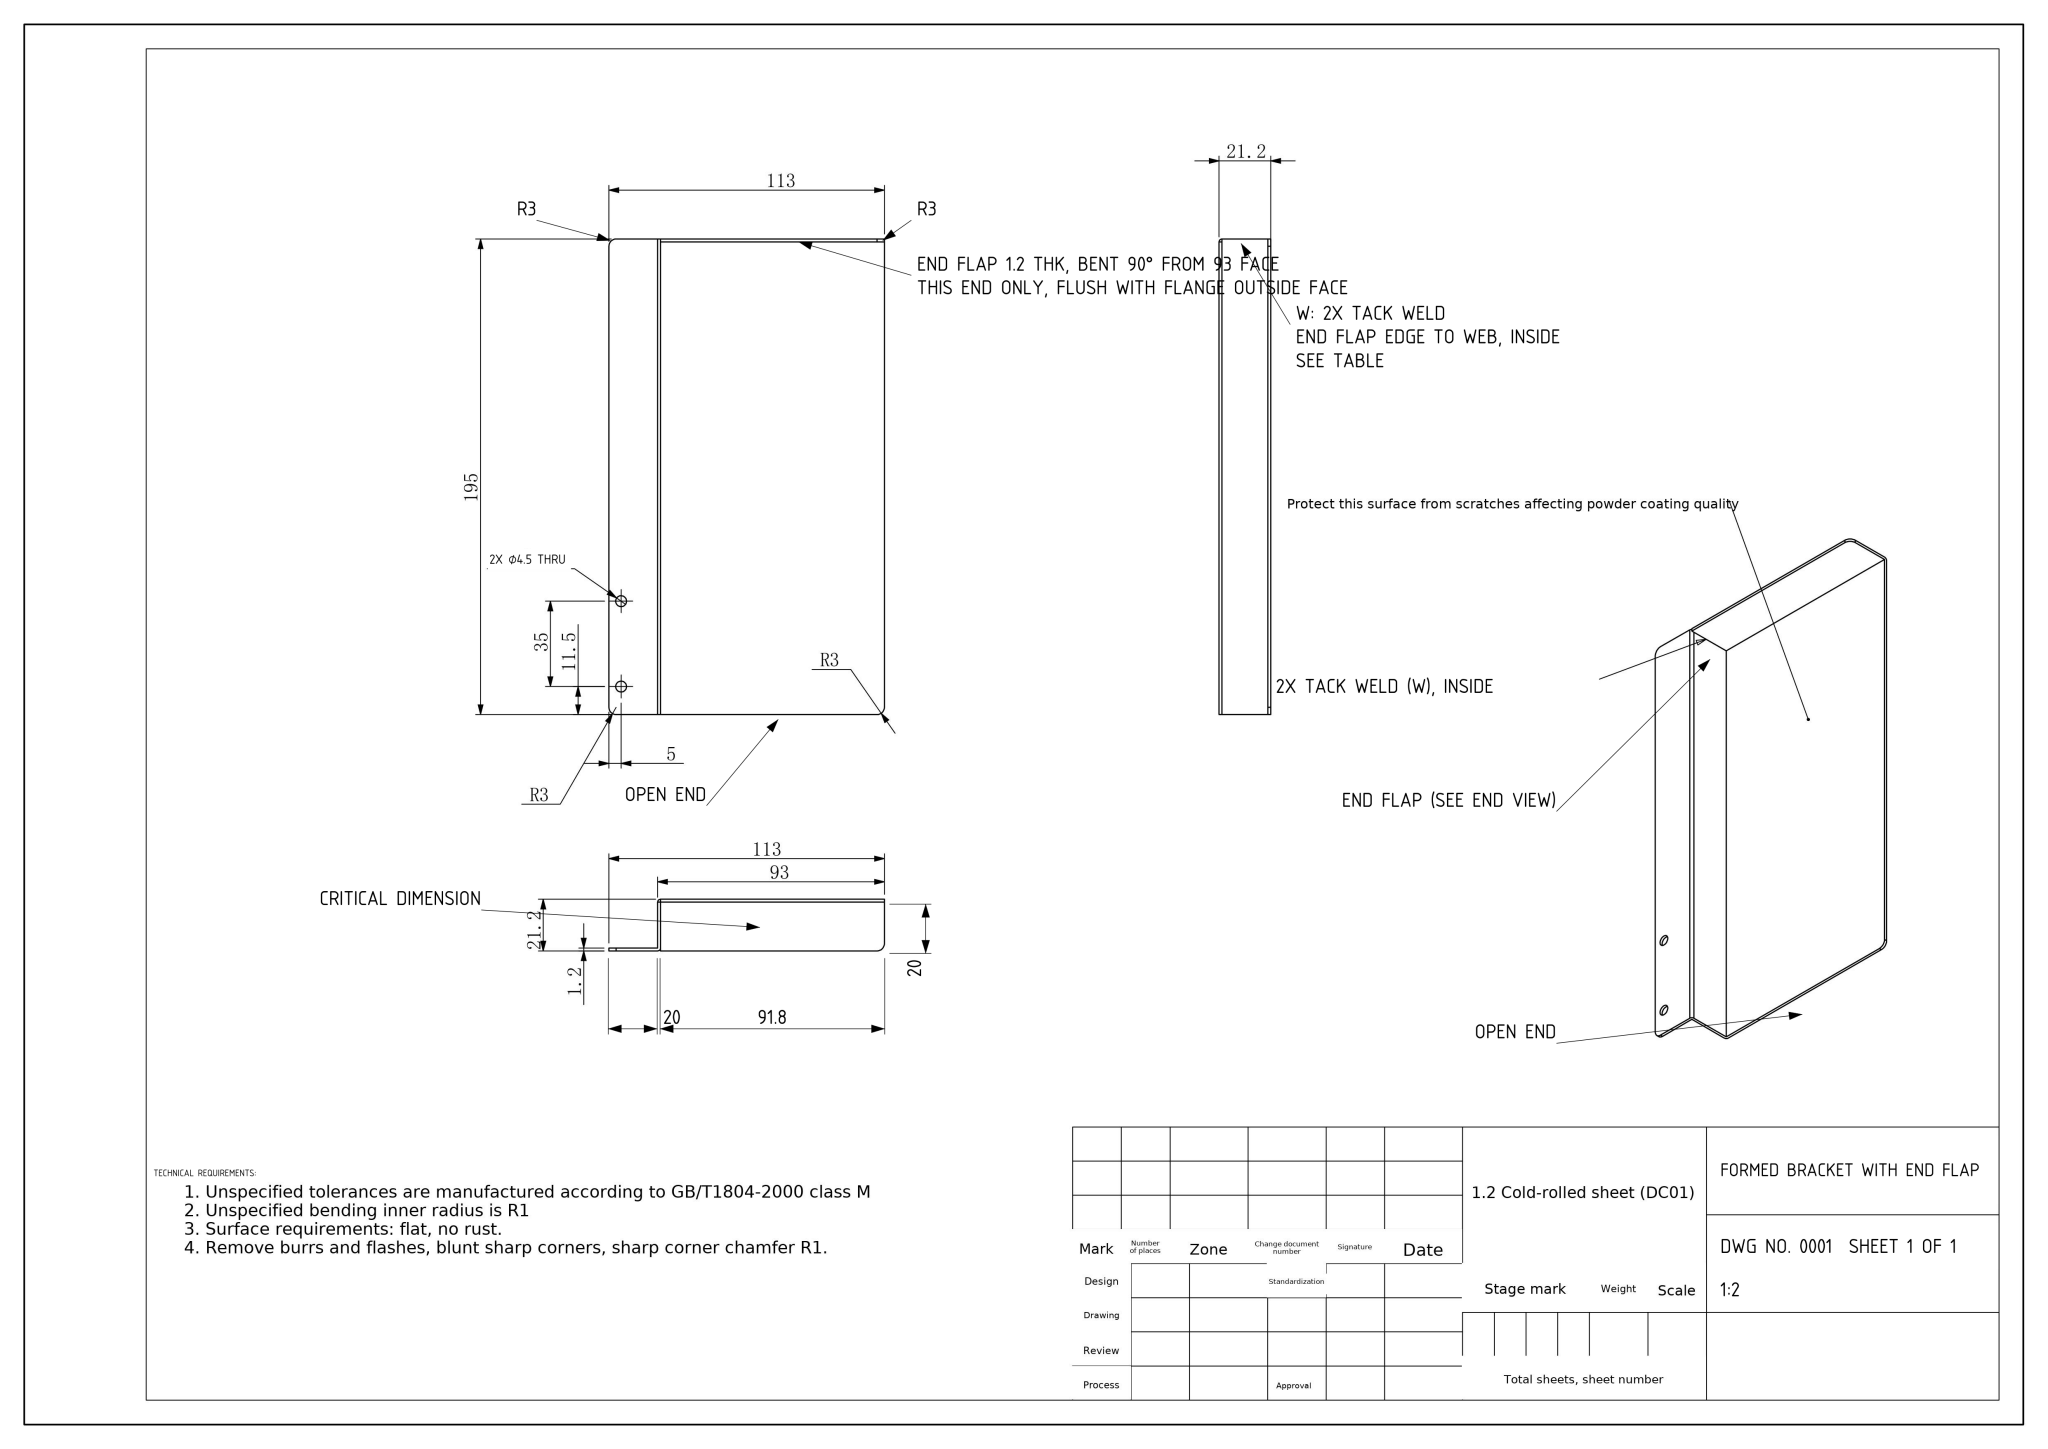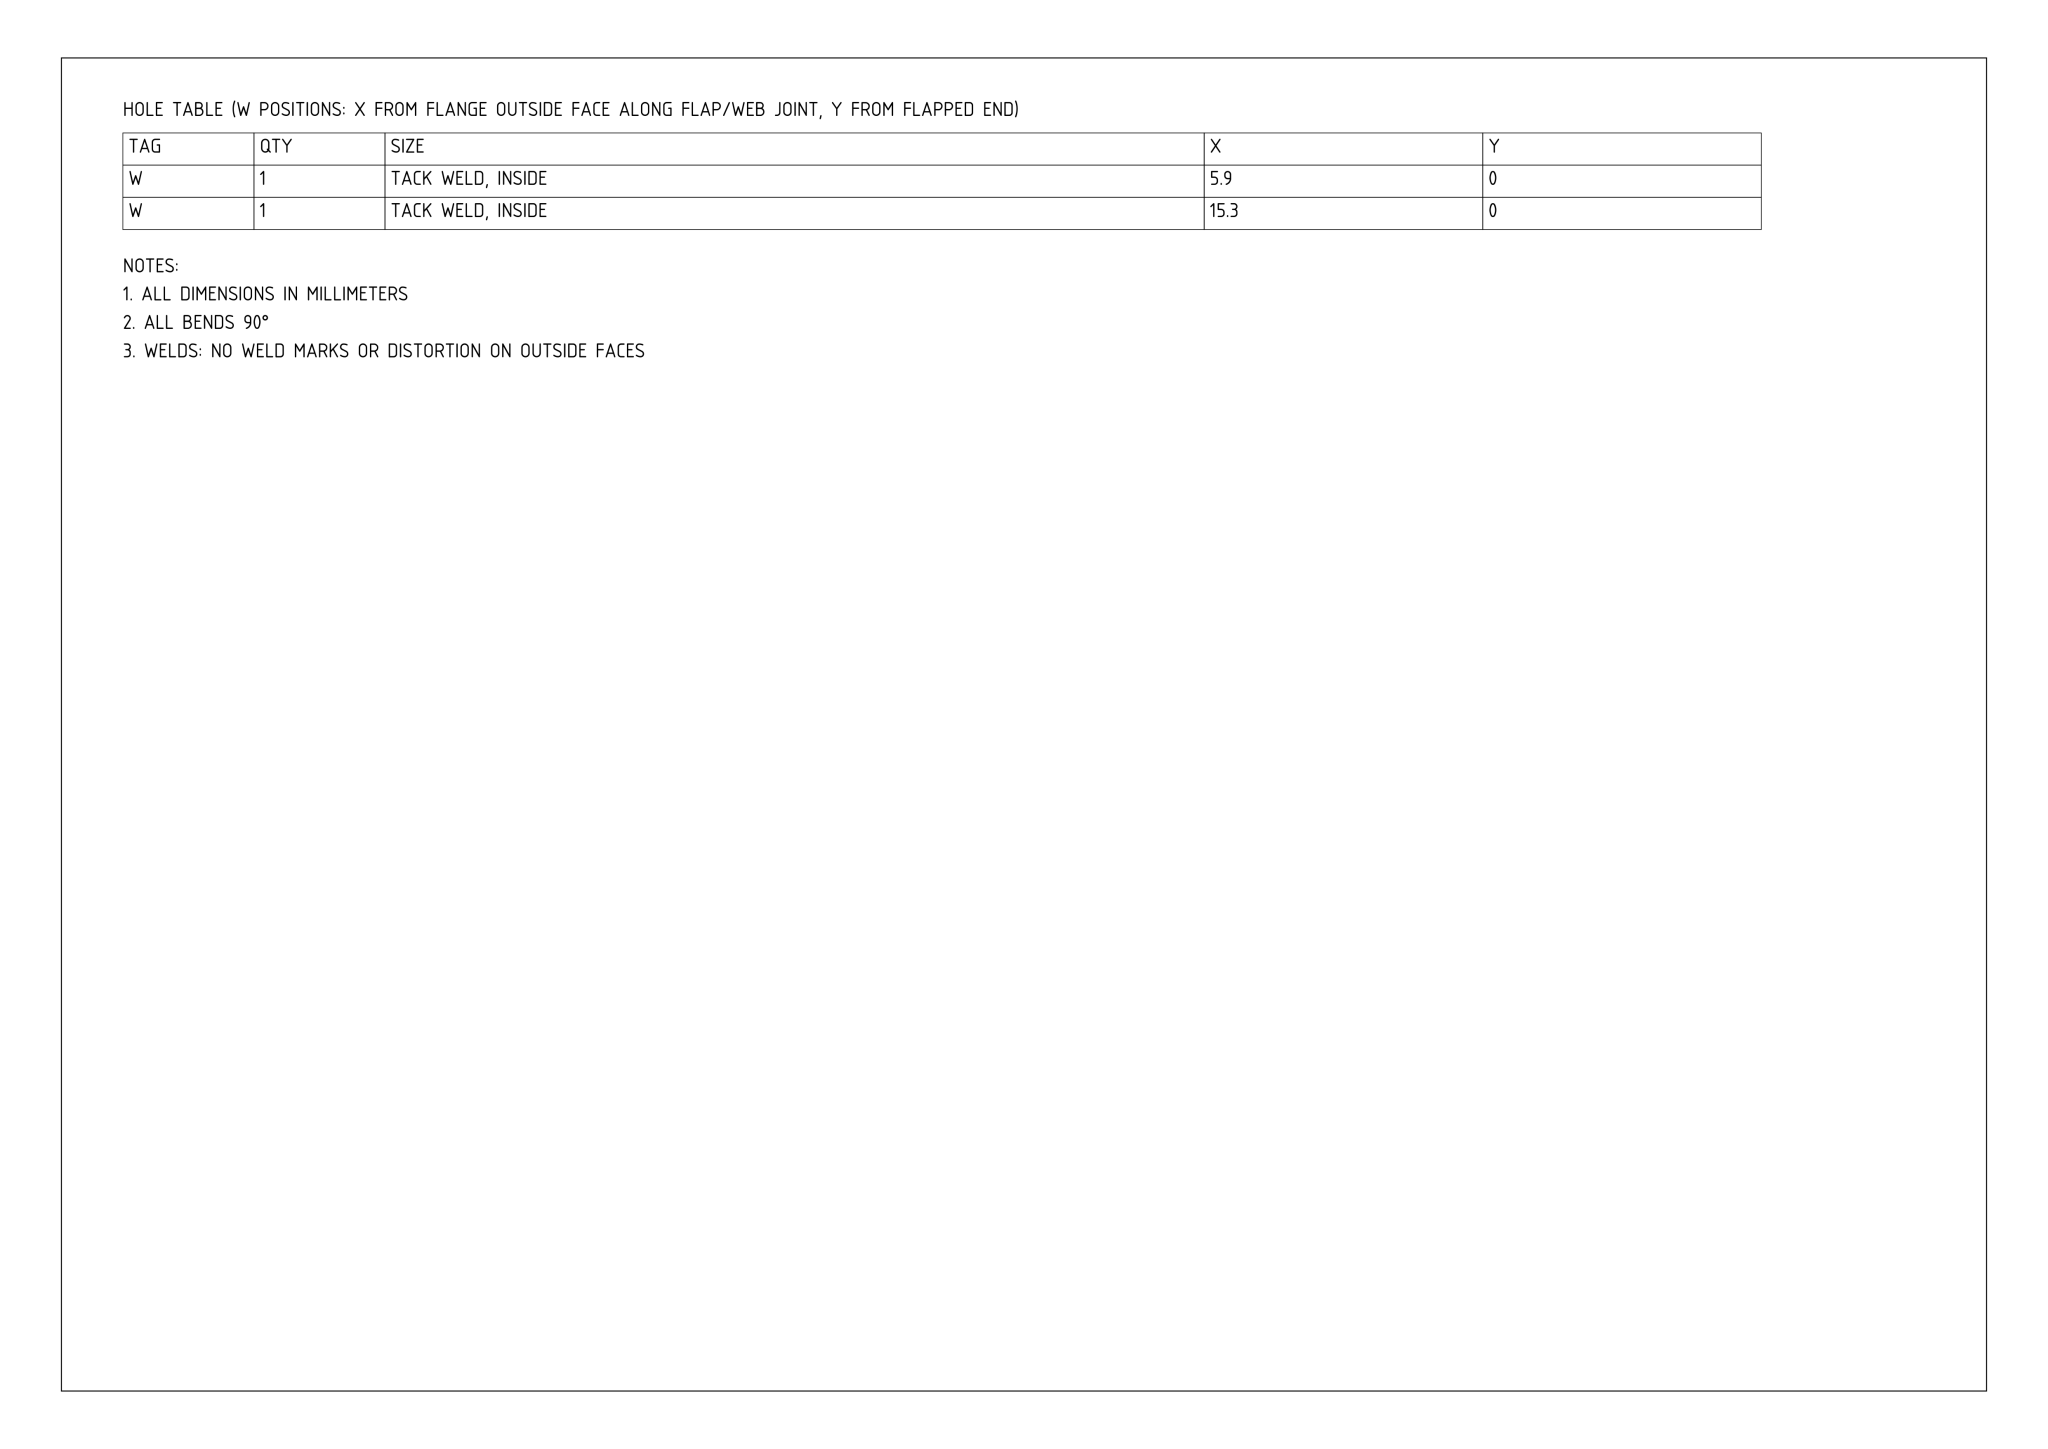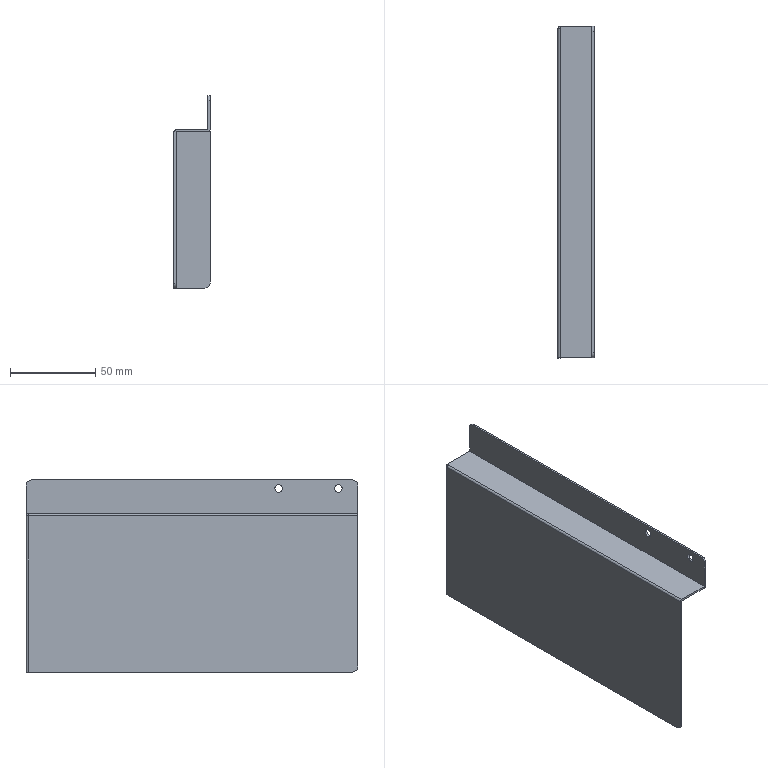Part | NX | mm | 1 solid | 30 faces | box 21.2 x 195 x 113 mm | volume 33127 mm3 | plane 16 | cylinder 14 | commonest cylinder face diameters 4.5 x4 6 x4 2.404 x3 0.004 x3